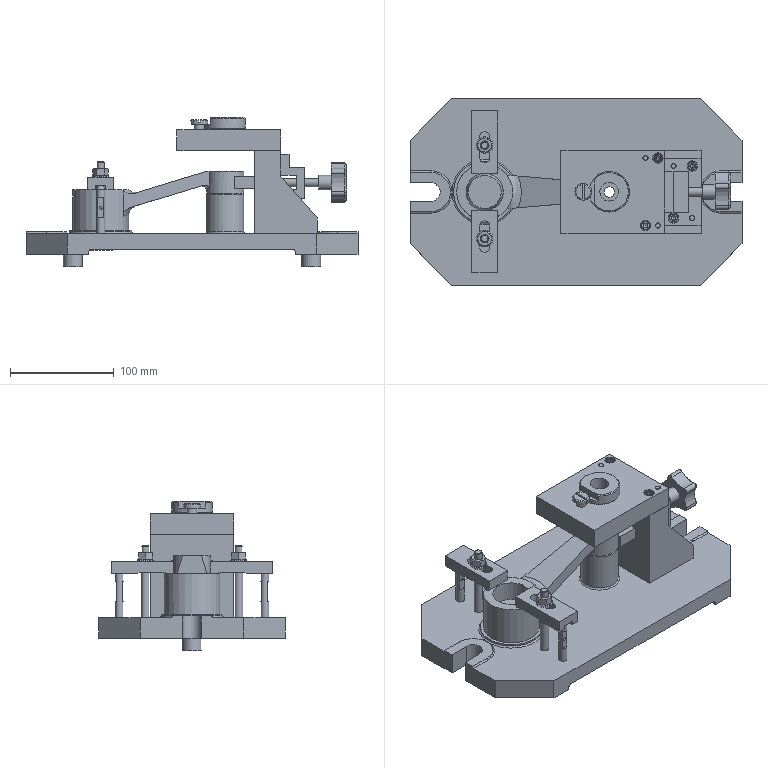Assembly | NX | mm | 37 component files | 37 solids | 688 faces | box 320 x 180 x 144 mm | volume 1502491 mm3 | plane 359 | cone 159 | cylinder 138 | torus 24 | spline 5 | sphere 3 | commonest cylinder face diameters 5 x22 8 x16 10 x15 6 x10 5.5 x10 4.826 x10 8.5 x10 3 x6
Bill of materials:
GB-T70.1-2000,M5x10 | 2 |  | Hexagon Socket Head Cap Screw, GB-T 70.1-2000,M5x10
unnamed part 1 | 1 |  | Rectangular block with a stepped Z/S-shaped side profile: two offset outer flanges joined by a thicker central section, with four small through holes in the flanges and one larger central through hole.
unnamed part 2 | 1 |  | Lever-like arm: a large cylindrical boss with a big through bore, joined by a tapered, inclined web to a smaller cylindrical boss with a small through hole. The two bosses sit at different heights.
GB-T6170_F-2000,M8x1.25 | 2 |  | Hexagonal prism with a central round through bore. Both ends are chamfered at the corners, and the bore entry is chamfered.
unnamed part 3 | 1 |  | Flat rectangular plate with a V-shaped notch on one edge ending in a small rectangular relief slot at the apex. The opposite edge has an open-ended slot with a rounded inner end.
unnamed part 4 | 1 |  | Stepped, slotted-head pin or screw: a chamfered round head with a straight slot across it, a cylindrical shoulder of smaller diameter, a reduced neck or undercut, and a smaller cylindrical shank with a chamfered end.
GB-T70.1-2000,M5x12 | 4 |  | Hexagon Socket Head Cap Screw, GB-T 70.1-2000,M5x12
unnamed part 5 | 1 |  | L-shaped angle bracket: a vertical wall on a base plate, braced by two triangular side gussets. The wall has a rectangular through window and several holes, and the top face and base also carry holes, including one larger counterbored hole in the base.
unnamed part 6 | 2 |  | Thick cylindrical ring or spacer with a central round through hole and flat ends.
unnamed part 7 | 1 |  | Five-lobed star-shaped knob with chamfered edges, a short cylindrical hub, and a long slender shaft. Near the tip the shaft has a reduced groove, and the end is rounded.
unnamed part 8 | 2 |  | Stepped cylindrical pin with a longer main diameter, a shorter reduced-diameter end section, and chamfered ends.
unnamed part 9 | 1 |  | Flanged bushing: a cylindrical body with a central through bore and a larger flange at one end. The flange has a single flat (D-cut) on one side, and the outer edges are chamfered.
unnamed part 10 | 4 |  | Plain solid cylindrical pin with chamfered ends.
unnamed part 11 | 2 |  | Rectangular block with an elongated obround through slot along its length. The underside has a shallow recessed channel with chamfered transitions, leaving a narrow foot at one end and a wider land at the other.
unnamed part 12 | 1 |  | Short thick-walled cylindrical ring or sleeve: plain cylindrical outside, a concentric through bore, flat end faces, and small chamfers on the outer edges at both ends.
unnamed part 13 | 2 |  | Slender cylindrical pin with a domed (rounded) end and a chamfered opposite end. Partway along it has a section with two opposite flats, and a small through hole crosses the pin through that flatted section.
GB-T97_2-2002,M8 | 2 |  | Thin flat annular ring (washer-like disc) with a single concentric through-hole and a chamfer around the outer edge of one face.
unnamed part 14 | 1 |  | Stepped cylindrical solid with a large head and a smaller shank. The head has a flat top face and a chamfered top edge, with a thin shoulder step under it. The shank has a short reduced-diameter neck or relief groove next to the head and a chamfered bottom end.
GB-T70.1-2000,M5x20 | 4 |  | Hexagon Socket Head Cap Screw, GB-T 70.1-2000,M5x20
unnamed part 15 | 1 |  | Rectangular flat block or plate with one large through bore, placed off-center. Four smaller through holes sit in two pairs along one edge, and the isometric view suggests two of them are counterbored. One small blind hole with a conical bottom sits on the other side of the large bore.
unnamed part 16 | 1 |  | Elongated plate with chamfered corners, which gives an octagonal outline. It has open U-shaped slots at both short ends with shallow recessed or spot-faced areas around them. There is a shallow raised or recessed annular pad with a through hole on one side, and a tubular cylindrical boss with a through bore near the center. Small holes are arranged in a line of four on one side and a rectangular group of four on the other. The underside appears relieved between thicker end pads.
Mates:
1. fix | fixture_body 1 component
2. concentric | cyl_loc_pin 1 edge | fixture_body 1 edge
3. concentric | part_drawing 1 edge | fixture_body 1 edge
4. touch align | drill_jig_support 1 face | fixture_body 1 face
5. touch align | drill_jig_plate 1 face | drill_jig_support 1 face
6. touch align | drill_jig_plate 1 face | drill_jig_support 1 face
7. concentric | drill_jig_support 1 edge | fixture_body 1 arc
8. concentric | bushing 1 edge | drill_jig_plate 1 edge
9. concentric | drill_bush_screw 1 edge | drill_jig_plate 1 arc
10. touch align | mov_v_block 1 face | drill_jig_support 1 face
11. touch align | mov_v_block 1 face | drill_jig_support 1 face
12. touch align | part_drawing 1 face | mov_v_block 1 face
13. touch align | part_drawing 1 face | fixture_body 1 face
14. touch align | clamp_support 1 face | drill_jig_support 1 face
15. concentric | clamp_support 1 edge | drill_jig_support 1 arc
16. touch align | hex_handle 1 face | clamp_support 1 face
17. touch align | hex_handle 1 face | mov_v_block 1 face
18. touch align | adj_support 2 face | fixture_body 1 face
19. touch align | mov_clamp_plate 2 face | adj_support 2 face
20. touch align | mov_clamp_plate 2 face | part_drawing 1 face
21. center | mov_clamp_plate 2 face | mov_clamp_plate 2 face | assembly datumplane
22. concentric | repl_drill_bush 1 edge | drill_jig_plate 1 edge
23. touch align | lg_adj_support 2 face | fixture_body 1 face
24. distance | lg_adj_support 2 face | mov_clamp_plate 2 face
25. distance | mov_clamp_plate 2 face | assembly datumplane
26. touch align | adj_support 1 face | fixture_body 1 face
27. touch align | lg_adj_support 1 face | fixture_body 1 face
28. distance | mov_clamp_plate 1 face | assembly datumplane
29. touch align | GB-T6170_F-2000_M8x1_25 2 face | lg_adj_support 2 face
30. touch align | GB-T97_2-2002_M8 2 face | lg_adj_support 2 face
31. touch align | GB-T97_2-2002_M8 2 face | mov_clamp_plate 2 face
32. touch align | GB-T6170_F-2000_M8x1_25 2 face | GB-T97_2-2002_M8 2 face
33. bond | mov_clamp_plate 1 component | assembly component
34. bond | GB-T97_2-2002_M8 2 component | assembly component
35. bond | GB-T6170_F-2000_M8x1_25 2 component | assembly component
36. bond | GB-T97_2-2002_M8 1 component | assembly component
37. bond | GB-T6170_F-2000_M8x1_25 1 component | assembly component
38. linear | assembly datumaxis | assembly cartesiancoordinatesystem | assembly cartesiancoordinatesystem
39. linear | assembly datumaxis | assembly cartesiancoordinatesystem | assembly cartesiancoordinatesystem
40. concentric | dowel_pin 4 edge | drill_jig_plate 1 edge
41. concentric | dowel_pin 3 edge | drill_jig_plate 1 edge
42. concentric | GB-T70_1-2000_M5x20 3 edge | drill_jig_plate 1 edge
43. concentric | GB-T70_1-2000_M5x20 4 edge | drill_jig_plate 1 edge
44. concentric | dowel_pin 1 edge | drill_jig_support 1 edge
45. concentric | dowel_pin 2 edge | drill_jig_support 1 edge
46. concentric | GB-T70_1-2000_M5x20 2 edge | drill_jig_support 1 edge
47. concentric | GB-T70_1-2000_M5x20 1 edge | drill_jig_support 1 edge
48. concentric | GB-T70_1-2000_M5x12 1 edge | clamp_support 1 edge
49. concentric | GB-T70_1-2000_M5x12 2 edge | clamp_support 1 edge
50. concentric | GB-T70_1-2000_M5x12 3 edge | clamp_support 1 edge
51. concentric | GB-T70_1-2000_M5x12 4 edge | clamp_support 1 edge
52. concentric | base_loc_block 2 edge | fixture_body 1 arc
53. concentric | base_loc_block 1 edge | fixture_body 1 arc
54. concentric | GB-T70_1-2000_M5x10 1 edge | base_loc_block 1 edge